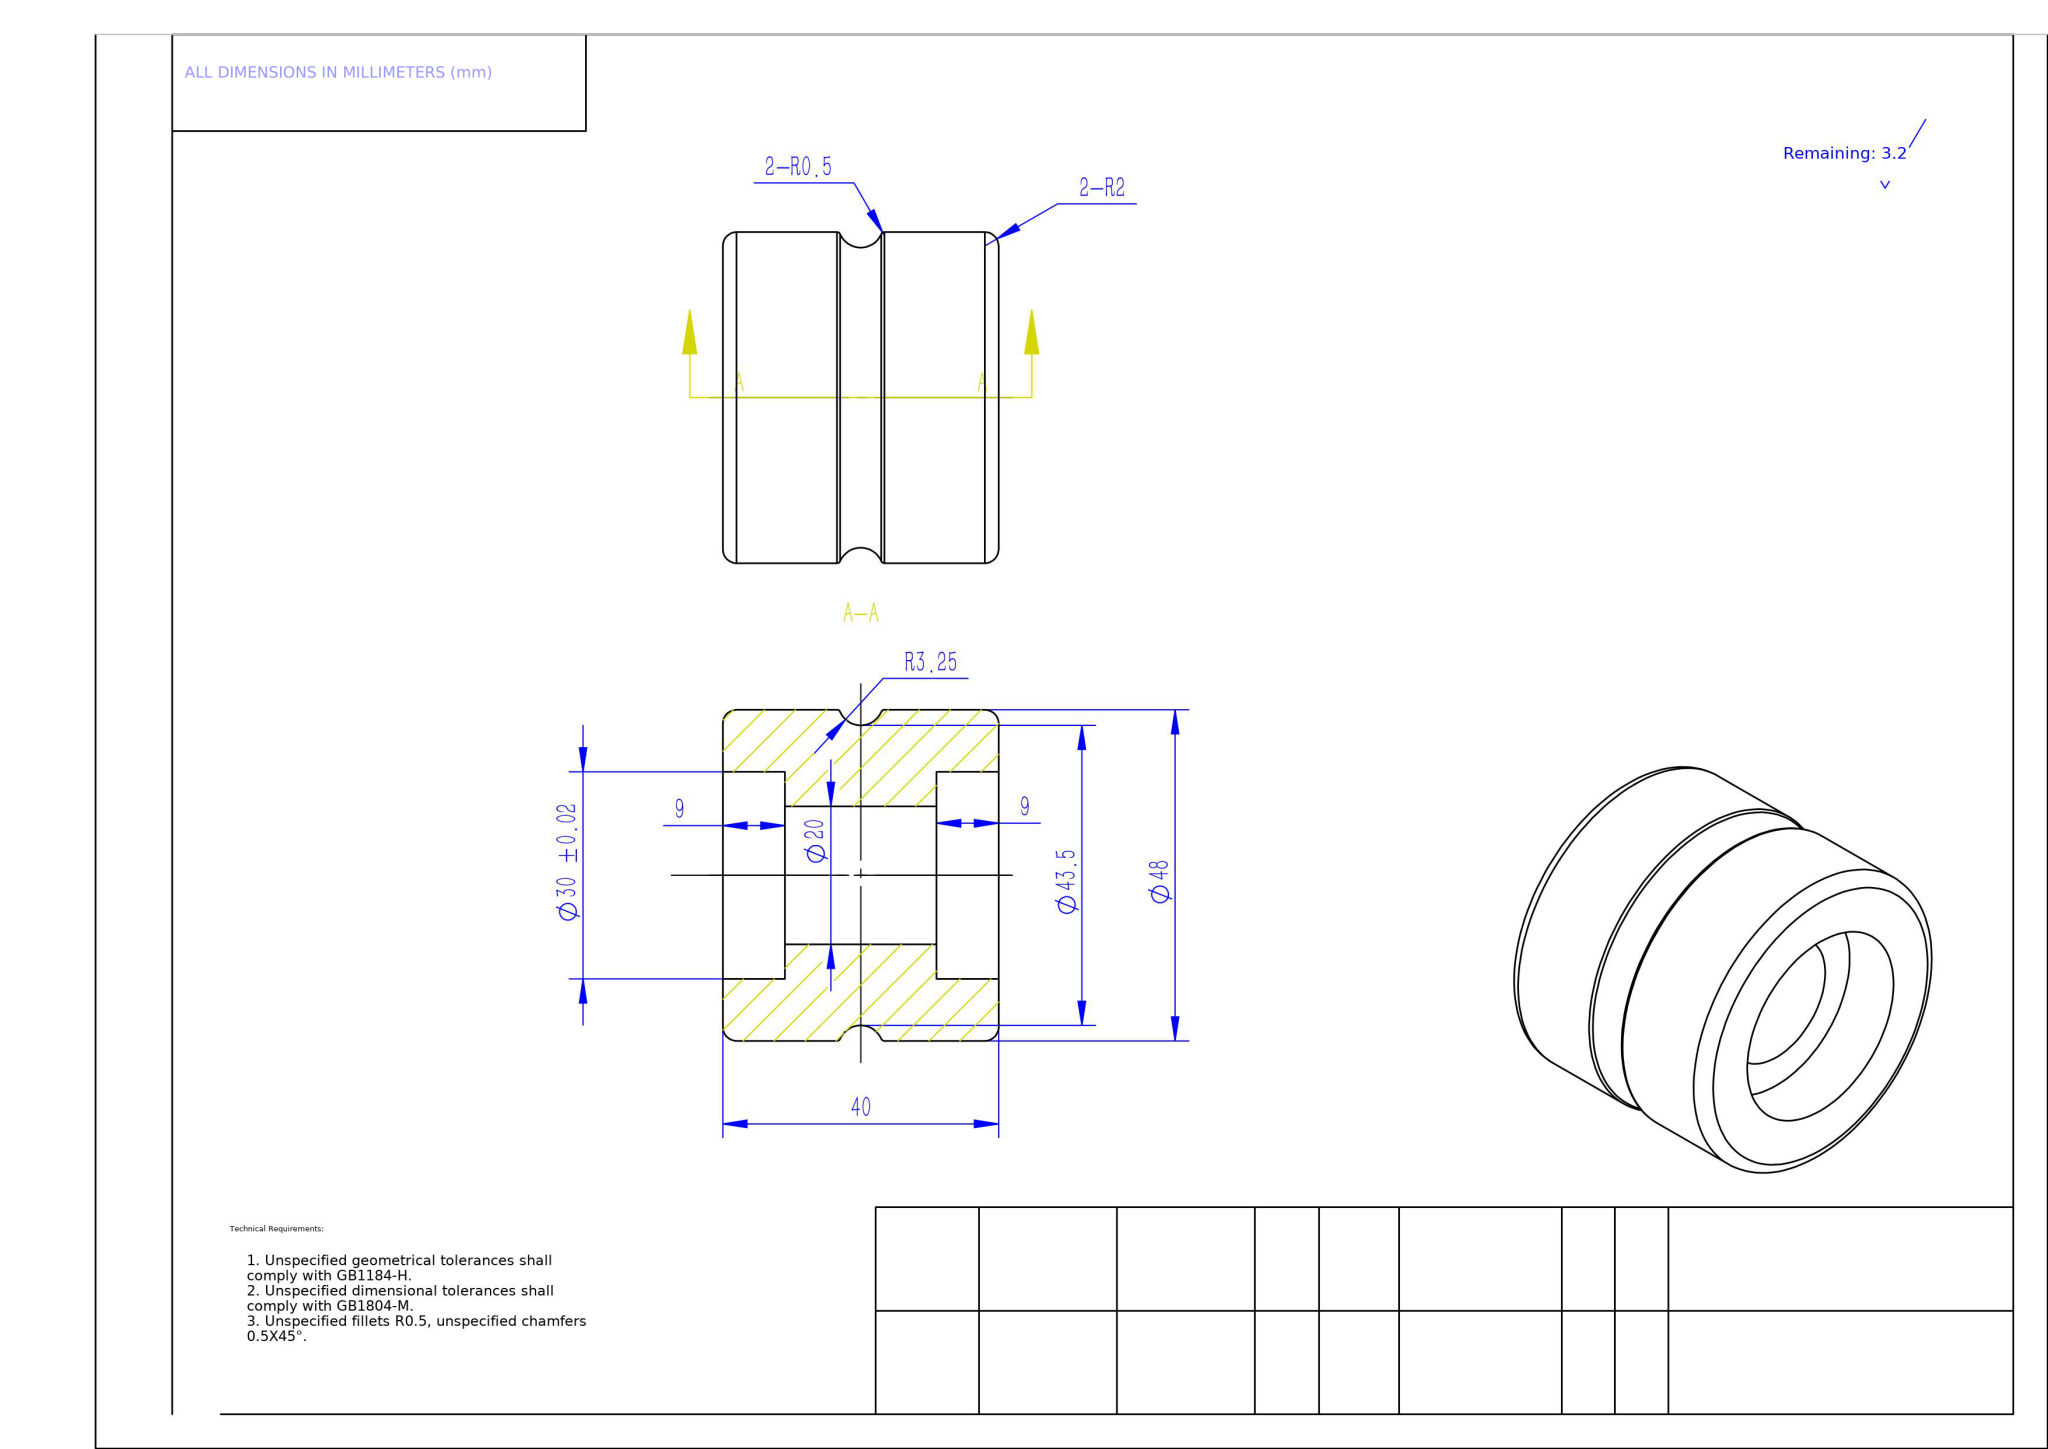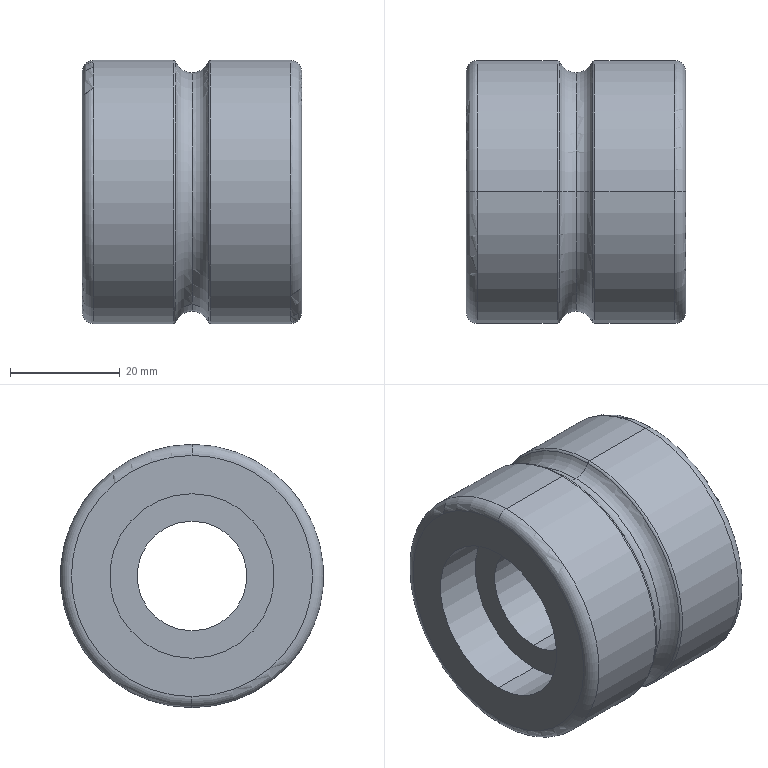Part | NX | mm | 1 solid | 26 faces | box 40 x 48 x 48 mm | volume 51009 mm3 | torus 12 | cylinder 10 | plane 4 | commonest cylinder face diameters 30 x4 48 x4 20 x2
STEP:
#1=COLOUR_RGB('',0.5294,0.549,0.549);
#2=FILL_AREA_STYLE_COLOUR('',#1);
#3=FILL_AREA_STYLE('',(#2));
#4=SURFACE_STYLE_FILL_AREA(#3);
#5=SURFACE_SIDE_STYLE('',(#4));
#6=SURFACE_STYLE_USAGE(.BOTH.,#5);
#7=PRESENTATION_STYLE_ASSIGNMENT((#6));
#8=CARTESIAN_POINT('',(17.021,0.,23.7));
#9=VERTEX_POINT('',#8);
#10=CARTESIAN_POINT('',(20.,0.,21.75));
#11=VERTEX_POINT('',#10);
#12=CARTESIAN_POINT('',(20.,0.,25.));
#13=DIRECTION('',(0.,-1.,0.));
#14=DIRECTION('',(0.,0.,-1.));
#15=AXIS2_PLACEMENT_3D('',#12,#13,#14);
#16=CIRCLE('',#15,3.25);
#17=EDGE_CURVE('',#9,#11,#16,.T.);
#18=ORIENTED_EDGE('',*,*,#17,.T.);
#19=CARTESIAN_POINT('',(20.,0.,-21.75));
#20=VERTEX_POINT('',#19);
#21=CARTESIAN_POINT('',(20.,0.,0.));
#22=DIRECTION('',(-1.,0.,0.));
#23=DIRECTION('',(0.,0.,1.));
#24=AXIS2_PLACEMENT_3D('',#21,#22,#23);
#25=CIRCLE('',#24,21.75);
#26=EDGE_CURVE('',#11,#20,#25,.T.);
#27=ORIENTED_EDGE('',*,*,#26,.T.);
#28=CARTESIAN_POINT('',(17.021,0.,-23.7));
#29=VERTEX_POINT('',#28);
#30=CARTESIAN_POINT('',(20.,0.,-25.));
#31=DIRECTION('',(0.,1.,0.));
#32=DIRECTION('',(0.,-0.,1.));
#33=AXIS2_PLACEMENT_3D('',#30,#31,#32);
#34=CIRCLE('',#33,3.25);
#35=EDGE_CURVE('',#29,#20,#34,.T.);
#36=ORIENTED_EDGE('',*,*,#35,.F.);
#37=CARTESIAN_POINT('',(17.021,0.,0.));
#38=DIRECTION('',(1.,0.,0.));
#39=DIRECTION('',(0.,0.,-1.));
#40=AXIS2_PLACEMENT_3D('',#37,#38,#39);
#41=CIRCLE('',#40,23.7);
#42=EDGE_CURVE('',#29,#9,#41,.T.);
#43=ORIENTED_EDGE('',*,*,#42,.T.);
#44=EDGE_LOOP('',(#18,#27,#36,#43));
#45=FACE_OUTER_BOUND('',#44,.T.);
#46=CARTESIAN_POINT('',(20.,0.,0.));
#47=DIRECTION('',(-1.,0.,0.));
#48=DIRECTION('',(0.,0.,1.));
#49=AXIS2_PLACEMENT_3D('',#46,#47,#48);
#50=TOROIDAL_SURFACE('',#49,25.,3.25);
#51=ADVANCED_FACE('',(#45),#50,.F.);
#52=ORIENTED_EDGE('',*,*,#35,.T.);
#53=CARTESIAN_POINT('',(20.,0.,0.));
#54=DIRECTION('',(-1.,0.,0.));
#55=DIRECTION('',(0.,0.,1.));
#56=AXIS2_PLACEMENT_3D('',#53,#54,#55);
#57=CIRCLE('',#56,21.75);
#58=EDGE_CURVE('',#20,#11,#57,.T.);
#59=ORIENTED_EDGE('',*,*,#58,.T.);
#60=ORIENTED_EDGE('',*,*,#17,.F.);
#61=CARTESIAN_POINT('',(17.021,0.,0.));
#62=DIRECTION('',(1.,0.,0.));
#63=DIRECTION('',(0.,0.,-1.));
#64=AXIS2_PLACEMENT_3D('',#61,#62,#63);
#65=CIRCLE('',#64,23.7);
#66=EDGE_CURVE('',#9,#29,#65,.T.);
#67=ORIENTED_EDGE('',*,*,#66,.T.);
#68=EDGE_LOOP('',(#52,#59,#60,#67));
#69=FACE_OUTER_BOUND('',#68,.T.);
#70=CARTESIAN_POINT('',(20.,0.,0.));
#71=DIRECTION('',(-1.,0.,0.));
#72=DIRECTION('',(0.,0.,1.));
#73=AXIS2_PLACEMENT_3D('',#70,#71,#72);
#74=TOROIDAL_SURFACE('',#73,25.,3.25);
#75=ADVANCED_FACE('',(#69),#74,.F.);
#76=CARTESIAN_POINT('',(16.563,0.,24.));
#77=VERTEX_POINT('',#76);
#78=CARTESIAN_POINT('',(16.563,0.,-24.));
#79=VERTEX_POINT('',#78);
#80=CARTESIAN_POINT('',(16.563,0.,0.));
#81=DIRECTION('',(-1.,0.,0.));
#82=DIRECTION('',(0.,0.,-1.));
#83=AXIS2_PLACEMENT_3D('',#80,#81,#82);
#84=CIRCLE('',#83,24.);
#85=EDGE_CURVE('',#77,#79,#84,.T.);
#86=ORIENTED_EDGE('',*,*,#85,.F.);
#87=CARTESIAN_POINT('',(16.563,0.,23.5));
#88=DIRECTION('',(0.,1.,-0.));
#89=DIRECTION('',(0.,0.,1.));
#90=AXIS2_PLACEMENT_3D('',#87,#88,#89);
#91=CIRCLE('',#90,0.5);
#92=EDGE_CURVE('',#77,#9,#91,.T.);
#93=ORIENTED_EDGE('',*,*,#92,.T.);
#94=ORIENTED_EDGE('',*,*,#42,.F.);
#95=CARTESIAN_POINT('',(16.563,0.,-23.5));
#96=DIRECTION('',(0.,-1.,0.));
#97=DIRECTION('',(0.,0.,-1.));
#98=AXIS2_PLACEMENT_3D('',#95,#96,#97);
#99=CIRCLE('',#98,0.5);
#100=EDGE_CURVE('',#79,#29,#99,.T.);
#101=ORIENTED_EDGE('',*,*,#100,.F.);
#102=EDGE_LOOP('',(#86,#93,#94,#101));
#103=FACE_OUTER_BOUND('',#102,.T.);
#104=CARTESIAN_POINT('',(16.563,0.,0.));
#105=DIRECTION('',(1.,0.,0.));
#106=DIRECTION('',(0.,0.,-1.));
#107=AXIS2_PLACEMENT_3D('',#104,#105,#106);
#108=TOROIDAL_SURFACE('',#107,23.5,0.5);
#109=ADVANCED_FACE('',(#103),#108,.T.);
#110=CARTESIAN_POINT('',(22.979,0.,23.7));
#111=VERTEX_POINT('',#110);
#112=CARTESIAN_POINT('',(22.979,0.,-23.7));
#113=VERTEX_POINT('',#112);
#114=CARTESIAN_POINT('',(22.979,0.,0.));
#115=DIRECTION('',(-1.,0.,0.));
#116=DIRECTION('',(0.,0.,1.));
#117=AXIS2_PLACEMENT_3D('',#114,#115,#116);
#118=CIRCLE('',#117,23.7);
#119=EDGE_CURVE('',#111,#113,#118,.T.);
#120=ORIENTED_EDGE('',*,*,#119,.F.);
#121=CARTESIAN_POINT('',(23.437,0.,24.));
#122=VERTEX_POINT('',#121);
#123=CARTESIAN_POINT('',(23.437,0.,23.5));
#124=DIRECTION('',(0.,1.,-0.));
#125=DIRECTION('',(0.,0.,1.));
#126=AXIS2_PLACEMENT_3D('',#123,#124,#125);
#127=CIRCLE('',#126,0.5);
#128=EDGE_CURVE('',#111,#122,#127,.T.);
#129=ORIENTED_EDGE('',*,*,#128,.T.);
#130=CARTESIAN_POINT('',(23.437,0.,-24.));
#131=VERTEX_POINT('',#130);
#132=CARTESIAN_POINT('',(23.437,0.,0.));
#133=DIRECTION('',(1.,0.,0.));
#134=DIRECTION('',(0.,0.,-1.));
#135=AXIS2_PLACEMENT_3D('',#132,#133,#134);
#136=CIRCLE('',#135,24.);
#137=EDGE_CURVE('',#131,#122,#136,.T.);
#138=ORIENTED_EDGE('',*,*,#137,.F.);
#139=CARTESIAN_POINT('',(23.437,0.,-23.5));
#140=DIRECTION('',(0.,-1.,0.));
#141=DIRECTION('',(0.,0.,-1.));
#142=AXIS2_PLACEMENT_3D('',#139,#140,#141);
#143=CIRCLE('',#142,0.5);
#144=EDGE_CURVE('',#113,#131,#143,.T.);
#145=ORIENTED_EDGE('',*,*,#144,.F.);
#146=EDGE_LOOP('',(#120,#129,#138,#145));
#147=FACE_OUTER_BOUND('',#146,.T.);
#148=CARTESIAN_POINT('',(23.437,0.,0.));
#149=DIRECTION('',(1.,0.,0.));
#150=DIRECTION('',(0.,0.,-1.));
#151=AXIS2_PLACEMENT_3D('',#148,#149,#150);
#152=TOROIDAL_SURFACE('',#151,23.5,0.5);
#153=ADVANCED_FACE('',(#147),#152,.T.);
#154=CARTESIAN_POINT('',(2.,0.,-24.));
#155=VERTEX_POINT('',#154);
#156=CARTESIAN_POINT('',(2.,0.,24.));
#157=VERTEX_POINT('',#156);
#158=CARTESIAN_POINT('',(2.,0.,0.));
#159=DIRECTION('',(1.,0.,0.));
#160=DIRECTION('',(0.,0.,1.));
#161=AXIS2_PLACEMENT_3D('',#158,#159,#160);
#162=CIRCLE('',#161,24.);
#163=EDGE_CURVE('',#155,#157,#162,.T.);
#164=ORIENTED_EDGE('',*,*,#163,.F.);
#165=CARTESIAN_POINT('',(-0.,0.,-22.));
#166=VERTEX_POINT('',#165);
#167=CARTESIAN_POINT('',(2.,0.,-22.));
#168=DIRECTION('',(0.,1.,0.));
#169=DIRECTION('',(0.,-0.,1.));
#170=AXIS2_PLACEMENT_3D('',#167,#168,#169);
#171=CIRCLE('',#170,2.);
#172=EDGE_CURVE('',#155,#166,#171,.T.);
#173=ORIENTED_EDGE('',*,*,#172,.T.);
#174=CARTESIAN_POINT('',(-0.,0.,22.));
#175=VERTEX_POINT('',#174);
#176=CARTESIAN_POINT('',(-0.,0.,0.));
#177=DIRECTION('',(-1.,0.,0.));
#178=DIRECTION('',(0.,0.,1.));
#179=AXIS2_PLACEMENT_3D('',#176,#177,#178);
#180=CIRCLE('',#179,22.);
#181=EDGE_CURVE('',#175,#166,#180,.T.);
#182=ORIENTED_EDGE('',*,*,#181,.F.);
#183=CARTESIAN_POINT('',(2.,0.,22.));
#184=DIRECTION('',(0.,-1.,0.));
#185=DIRECTION('',(0.,0.,-1.));
#186=AXIS2_PLACEMENT_3D('',#183,#184,#185);
#187=CIRCLE('',#186,2.);
#188=EDGE_CURVE('',#157,#175,#187,.T.);
#189=ORIENTED_EDGE('',*,*,#188,.F.);
#190=EDGE_LOOP('',(#164,#173,#182,#189));
#191=FACE_OUTER_BOUND('',#190,.T.);
#192=CARTESIAN_POINT('',(2.,0.,0.));
#193=DIRECTION('',(-1.,0.,0.));
#194=DIRECTION('',(0.,0.,1.));
#195=AXIS2_PLACEMENT_3D('',#192,#193,#194);
#196=TOROIDAL_SURFACE('',#195,22.,2.);
#197=ADVANCED_FACE('',(#191),#196,.T.);
#198=CARTESIAN_POINT('',(38.,0.,24.));
#199=VERTEX_POINT('',#198);
#200=CARTESIAN_POINT('',(38.,0.,-24.));
#201=VERTEX_POINT('',#200);
#202=CARTESIAN_POINT('',(38.,0.,0.));
#203=DIRECTION('',(-1.,0.,0.));
#204=DIRECTION('',(0.,0.,-1.));
#205=AXIS2_PLACEMENT_3D('',#202,#203,#204);
#206=CIRCLE('',#205,24.);
#207=EDGE_CURVE('',#199,#201,#206,.T.);
#208=ORIENTED_EDGE('',*,*,#207,.F.);
#209=CARTESIAN_POINT('',(40.,0.,22.));
#210=VERTEX_POINT('',#209);
#211=CARTESIAN_POINT('',(38.,0.,22.));
#212=DIRECTION('',(0.,1.,-0.));
#213=DIRECTION('',(0.,0.,1.));
#214=AXIS2_PLACEMENT_3D('',#211,#212,#213);
#215=CIRCLE('',#214,2.);
#216=EDGE_CURVE('',#199,#210,#215,.T.);
#217=ORIENTED_EDGE('',*,*,#216,.T.);
#218=CARTESIAN_POINT('',(40.,0.,-22.));
#219=VERTEX_POINT('',#218);
#220=CARTESIAN_POINT('',(40.,0.,0.));
#221=DIRECTION('',(1.,0.,0.));
#222=DIRECTION('',(0.,0.,-1.));
#223=AXIS2_PLACEMENT_3D('',#220,#221,#222);
#224=CIRCLE('',#223,22.);
#225=EDGE_CURVE('',#219,#210,#224,.T.);
#226=ORIENTED_EDGE('',*,*,#225,.F.);
#227=CARTESIAN_POINT('',(38.,0.,-22.));
#228=DIRECTION('',(0.,-1.,0.));
#229=DIRECTION('',(0.,0.,-1.));
#230=AXIS2_PLACEMENT_3D('',#227,#228,#229);
#231=CIRCLE('',#230,2.);
#232=EDGE_CURVE('',#201,#219,#231,.T.);
#233=ORIENTED_EDGE('',*,*,#232,.F.);
#234=EDGE_LOOP('',(#208,#217,#226,#233));
#235=FACE_OUTER_BOUND('',#234,.T.);
#236=CARTESIAN_POINT('',(38.,0.,0.));
#237=DIRECTION('',(1.,0.,0.));
#238=DIRECTION('',(0.,0.,-1.));
#239=AXIS2_PLACEMENT_3D('',#236,#237,#238);
#240=TOROIDAL_SURFACE('',#239,22.,2.);
#241=ADVANCED_FACE('',(#235),#240,.T.);
#242=CARTESIAN_POINT('',(40.,0.,-15.));
#243=VERTEX_POINT('',#242);
#244=CARTESIAN_POINT('',(40.,0.,15.));
#245=VERTEX_POINT('',#244);
#246=CARTESIAN_POINT('',(40.,0.,0.));
#247=DIRECTION('',(-1.,0.,0.));
#248=DIRECTION('',(0.,0.,1.));
#249=AXIS2_PLACEMENT_3D('',#246,#247,#248);
#250=CIRCLE('',#249,15.);
#251=EDGE_CURVE('',#243,#245,#250,.T.);
#252=ORIENTED_EDGE('',*,*,#251,.F.);
#253=CARTESIAN_POINT('',(31.,0.,-15.));
#254=VERTEX_POINT('',#253);
#255=CARTESIAN_POINT('',(0.,0.,-15.));
#256=DIRECTION('',(-1.,0.,0.));
#257=VECTOR('',#256,1000.);
#258=LINE('',#255,#257);
#259=EDGE_CURVE('',#243,#254,#258,.T.);
#260=ORIENTED_EDGE('',*,*,#259,.T.);
#261=CARTESIAN_POINT('',(31.,0.,15.));
#262=VERTEX_POINT('',#261);
#263=CARTESIAN_POINT('',(31.,0.,0.));
#264=DIRECTION('',(-1.,0.,0.));
#265=DIRECTION('',(0.,0.,1.));
#266=AXIS2_PLACEMENT_3D('',#263,#264,#265);
#267=CIRCLE('',#266,15.);
#268=EDGE_CURVE('',#254,#262,#267,.T.);
#269=ORIENTED_EDGE('',*,*,#268,.T.);
#270=CARTESIAN_POINT('',(0.,0.,15.));
#271=DIRECTION('',(-1.,0.,0.));
#272=VECTOR('',#271,1000.);
#273=LINE('',#270,#272);
#274=EDGE_CURVE('',#245,#262,#273,.T.);
#275=ORIENTED_EDGE('',*,*,#274,.F.);
#276=EDGE_LOOP('',(#252,#260,#269,#275));
#277=FACE_OUTER_BOUND('',#276,.T.);
#278=CARTESIAN_POINT('',(0.,0.,0.));
#279=DIRECTION('',(-1.,0.,0.));
#280=DIRECTION('',(0.,0.,1.));
#281=AXIS2_PLACEMENT_3D('',#278,#279,#280);
#282=CYLINDRICAL_SURFACE('',#281,15.);
#283=ADVANCED_FACE('',(#277),#282,.F.);
#284=CARTESIAN_POINT('',(31.,0.,-10.));
#285=VERTEX_POINT('',#284);
#286=CARTESIAN_POINT('',(31.,0.,10.));
#287=VERTEX_POINT('',#286);
#288=CARTESIAN_POINT('',(31.,0.,0.));
#289=DIRECTION('',(-1.,0.,0.));
#290=DIRECTION('',(0.,0.,1.));
#291=AXIS2_PLACEMENT_3D('',#288,#289,#290);
#292=CIRCLE('',#291,10.);
#293=EDGE_CURVE('',#285,#287,#292,.T.);
#294=ORIENTED_EDGE('',*,*,#293,.F.);
#295=CARTESIAN_POINT('',(9.,0.,-10.));
#296=VERTEX_POINT('',#295);
#297=CARTESIAN_POINT('',(0.,0.,-10.));
#298=DIRECTION('',(-1.,0.,0.));
#299=VECTOR('',#298,1000.);
#300=LINE('',#297,#299);
#301=EDGE_CURVE('',#285,#296,#300,.T.);
#302=ORIENTED_EDGE('',*,*,#301,.T.);
#303=CARTESIAN_POINT('',(9.,0.,10.));
#304=VERTEX_POINT('',#303);
#305=CARTESIAN_POINT('',(9.,0.,0.));
#306=DIRECTION('',(-1.,0.,0.));
#307=DIRECTION('',(0.,0.,1.));
#308=AXIS2_PLACEMENT_3D('',#305,#306,#307);
#309=CIRCLE('',#308,10.);
#310=EDGE_CURVE('',#296,#304,#309,.T.);
#311=ORIENTED_EDGE('',*,*,#310,.T.);
#312=CARTESIAN_POINT('',(0.,0.,10.));
#313=DIRECTION('',(-1.,0.,0.));
#314=VECTOR('',#313,1000.);
#315=LINE('',#312,#314);
#316=EDGE_CURVE('',#287,#304,#315,.T.);
#317=ORIENTED_EDGE('',*,*,#316,.F.);
#318=EDGE_LOOP('',(#294,#302,#311,#317));
#319=FACE_OUTER_BOUND('',#318,.T.);
#320=CARTESIAN_POINT('',(0.,0.,0.));
#321=DIRECTION('',(-1.,0.,0.));
#322=DIRECTION('',(0.,0.,1.));
#323=AXIS2_PLACEMENT_3D('',#320,#321,#322);
#324=CYLINDRICAL_SURFACE('',#323,10.);
#325=ADVANCED_FACE('',(#319),#324,.F.);
#326=CARTESIAN_POINT('',(9.,0.,-15.));
#327=VERTEX_POINT('',#326);
#328=CARTESIAN_POINT('',(9.,0.,15.));
#329=VERTEX_POINT('',#328);
#330=CARTESIAN_POINT('',(9.,0.,0.));
#331=DIRECTION('',(-1.,0.,0.));
#332=DIRECTION('',(0.,0.,1.));
#333=AXIS2_PLACEMENT_3D('',#330,#331,#332);
#334=CIRCLE('',#333,15.);
#335=EDGE_CURVE('',#327,#329,#334,.T.);
#336=ORIENTED_EDGE('',*,*,#335,.F.);
#337=CARTESIAN_POINT('',(0.,0.,-15.));
#338=VERTEX_POINT('',#337);
#339=CARTESIAN_POINT('',(0.,0.,-15.));
#340=DIRECTION('',(-1.,0.,0.));
#341=VECTOR('',#340,1000.);
#342=LINE('',#339,#341);
#343=EDGE_CURVE('',#327,#338,#342,.T.);
#344=ORIENTED_EDGE('',*,*,#343,.T.);
#345=CARTESIAN_POINT('',(0.,0.,15.));
#346=VERTEX_POINT('',#345);
#347=CARTESIAN_POINT('',(0.,0.,0.));
#348=DIRECTION('',(-1.,0.,0.));
#349=DIRECTION('',(0.,0.,1.));
#350=AXIS2_PLACEMENT_3D('',#347,#348,#349);
#351=CIRCLE('',#350,15.);
#352=EDGE_CURVE('',#338,#346,#351,.T.);
#353=ORIENTED_EDGE('',*,*,#352,.T.);
#354=CARTESIAN_POINT('',(0.,0.,15.));
#355=DIRECTION('',(-1.,0.,0.));
#356=VECTOR('',#355,1000.);
#357=LINE('',#354,#356);
#358=EDGE_CURVE('',#329,#346,#357,.T.);
#359=ORIENTED_EDGE('',*,*,#358,.F.);
#360=EDGE_LOOP('',(#336,#344,#353,#359));
#361=FACE_OUTER_BOUND('',#360,.T.);
#362=CARTESIAN_POINT('',(0.,0.,0.));
#363=DIRECTION('',(-1.,0.,0.));
#364=DIRECTION('',(0.,0.,1.));
#365=AXIS2_PLACEMENT_3D('',#362,#363,#364);
#366=CYLINDRICAL_SURFACE('',#365,15.);
#367=ADVANCED_FACE('',(#361),#366,.F.);
#368=ORIENTED_EDGE('',*,*,#85,.T.);
#369=CARTESIAN_POINT('',(0.,0.,-24.));
#370=DIRECTION('',(-1.,0.,0.));
#371=VECTOR('',#370,1000.);
#372=LINE('',#369,#371);
#373=EDGE_CURVE('',#79,#155,#372,.T.);
#374=ORIENTED_EDGE('',*,*,#373,.T.);
#375=ORIENTED_EDGE('',*,*,#163,.T.);
#376=CARTESIAN_POINT('',(0.,0.,24.));
#377=DIRECTION('',(-1.,0.,0.));
#378=VECTOR('',#377,1000.);
#379=LINE('',#376,#378);
#380=EDGE_CURVE('',#77,#157,#379,.T.);
#381=ORIENTED_EDGE('',*,*,#380,.F.);
#382=EDGE_LOOP('',(#368,#374,#375,#381));
#383=FACE_OUTER_BOUND('',#382,.T.);
#384=CARTESIAN_POINT('',(0.,0.,0.));
#385=DIRECTION('',(-1.,0.,0.));
#386=DIRECTION('',(0.,0.,1.));
#387=AXIS2_PLACEMENT_3D('',#384,#385,#386);
#388=CYLINDRICAL_SURFACE('',#387,24.);
#389=ADVANCED_FACE('',(#383),#388,.T.);
#390=ORIENTED_EDGE('',*,*,#58,.F.);
#391=CARTESIAN_POINT('',(20.,0.,-25.));
#392=DIRECTION('',(0.,1.,0.));
#393=DIRECTION('',(0.,-0.,1.));
#394=AXIS2_PLACEMENT_3D('',#391,#392,#393);
#395=CIRCLE('',#394,3.25);
#396=EDGE_CURVE('',#20,#113,#395,.T.);
#397=ORIENTED_EDGE('',*,*,#396,.T.);
#398=CARTESIAN_POINT('',(22.979,0.,0.));
#399=DIRECTION('',(-1.,0.,0.));
#400=DIRECTION('',(0.,0.,1.));
#401=AXIS2_PLACEMENT_3D('',#398,#399,#400);
#402=CIRCLE('',#401,23.7);
#403=EDGE_CURVE('',#113,#111,#402,.T.);
#404=ORIENTED_EDGE('',*,*,#403,.T.);
#405=CARTESIAN_POINT('',(20.,0.,25.));
#406=DIRECTION('',(0.,-1.,0.));
#407=DIRECTION('',(0.,0.,-1.));
#408=AXIS2_PLACEMENT_3D('',#405,#406,#407);
#409=CIRCLE('',#408,3.25);
#410=EDGE_CURVE('',#11,#111,#409,.T.);
#411=ORIENTED_EDGE('',*,*,#410,.F.);
#412=EDGE_LOOP('',(#390,#397,#404,#411));
#413=FACE_OUTER_BOUND('',#412,.T.);
#414=CARTESIAN_POINT('',(20.,0.,0.));
#415=DIRECTION('',(-1.,0.,0.));
#416=DIRECTION('',(0.,0.,1.));
#417=AXIS2_PLACEMENT_3D('',#414,#415,#416);
#418=TOROIDAL_SURFACE('',#417,25.,3.25);
#419=ADVANCED_FACE('',(#413),#418,.F.);
#420=ORIENTED_EDGE('',*,*,#207,.T.);
#421=CARTESIAN_POINT('',(0.,0.,-24.));
#422=DIRECTION('',(-1.,0.,0.));
#423=VECTOR('',#422,1000.);
#424=LINE('',#421,#423);
#425=EDGE_CURVE('',#201,#131,#424,.T.);
#426=ORIENTED_EDGE('',*,*,#425,.T.);
#427=ORIENTED_EDGE('',*,*,#137,.T.);
#428=CARTESIAN_POINT('',(0.,0.,24.));
#429=DIRECTION('',(-1.,0.,0.));
#430=VECTOR('',#429,1000.);
#431=LINE('',#428,#430);
#432=EDGE_CURVE('',#199,#122,#431,.T.);
#433=ORIENTED_EDGE('',*,*,#432,.F.);
#434=EDGE_LOOP('',(#420,#426,#427,#433));
#435=FACE_OUTER_BOUND('',#434,.T.);
#436=CARTESIAN_POINT('',(0.,0.,0.));
#437=DIRECTION('',(-1.,0.,0.));
#438=DIRECTION('',(0.,0.,1.));
#439=AXIS2_PLACEMENT_3D('',#436,#437,#438);
#440=CYLINDRICAL_SURFACE('',#439,24.);
#441=ADVANCED_FACE('',(#435),#440,.T.);
#442=ORIENTED_EDGE('',*,*,#425,.F.);
#443=CARTESIAN_POINT('',(38.,0.,0.));
#444=DIRECTION('',(-1.,0.,0.));
#445=DIRECTION('',(0.,0.,-1.));
#446=AXIS2_PLACEMENT_3D('',#443,#444,#445);
#447=CIRCLE('',#446,24.);
#448=EDGE_CURVE('',#201,#199,#447,.T.);
#449=ORIENTED_EDGE('',*,*,#448,.T.);
#450=ORIENTED_EDGE('',*,*,#432,.T.);
#451=CARTESIAN_POINT('',(23.437,0.,0.));
#452=DIRECTION('',(1.,0.,0.));
#453=DIRECTION('',(0.,0.,-1.));
#454=AXIS2_PLACEMENT_3D('',#451,#452,#453);
#455=CIRCLE('',#454,24.);
#456=EDGE_CURVE('',#122,#131,#455,.T.);
#457=ORIENTED_EDGE('',*,*,#456,.T.);
#458=EDGE_LOOP('',(#442,#449,#450,#457));
#459=FACE_OUTER_BOUND('',#458,.T.);
#460=CARTESIAN_POINT('',(0.,0.,0.));
#461=DIRECTION('',(-1.,0.,0.));
#462=DIRECTION('',(0.,0.,1.));
#463=AXIS2_PLACEMENT_3D('',#460,#461,#462);
#464=CYLINDRICAL_SURFACE('',#463,24.);
#465=ADVANCED_FACE('',(#459),#464,.T.);
#466=ORIENTED_EDGE('',*,*,#26,.F.);
#467=ORIENTED_EDGE('',*,*,#410,.T.);
#468=ORIENTED_EDGE('',*,*,#119,.T.);
#469=ORIENTED_EDGE('',*,*,#396,.F.);
#470=EDGE_LOOP('',(#466,#467,#468,#469));
#471=FACE_OUTER_BOUND('',#470,.T.);
#472=CARTESIAN_POINT('',(20.,0.,0.));
#473=DIRECTION('',(-1.,0.,0.));
#474=DIRECTION('',(0.,0.,1.));
#475=AXIS2_PLACEMENT_3D('',#472,#473,#474);
#476=TOROIDAL_SURFACE('',#475,25.,3.25);
#477=ADVANCED_FACE('',(#471),#476,.F.);
#478=ORIENTED_EDGE('',*,*,#373,.F.);
#479=CARTESIAN_POINT('',(16.563,0.,0.));
#480=DIRECTION('',(-1.,0.,0.));
#481=DIRECTION('',(0.,0.,-1.));
#482=AXIS2_PLACEMENT_3D('',#479,#480,#481);
#483=CIRCLE('',#482,24.);
#484=EDGE_CURVE('',#79,#77,#483,.T.);
#485=ORIENTED_EDGE('',*,*,#484,.T.);
#486=ORIENTED_EDGE('',*,*,#380,.T.);
#487=CARTESIAN_POINT('',(2.,0.,0.));
#488=DIRECTION('',(1.,0.,0.));
#489=DIRECTION('',(0.,0.,1.));
#490=AXIS2_PLACEMENT_3D('',#487,#488,#489);
#491=CIRCLE('',#490,24.);
#492=EDGE_CURVE('',#157,#155,#491,.T.);
#493=ORIENTED_EDGE('',*,*,#492,.T.);
#494=EDGE_LOOP('',(#478,#485,#486,#493));
#495=FACE_OUTER_BOUND('',#494,.T.);
#496=CARTESIAN_POINT('',(0.,0.,0.));
#497=DIRECTION('',(-1.,0.,0.));
#498=DIRECTION('',(0.,0.,1.));
#499=AXIS2_PLACEMENT_3D('',#496,#497,#498);
#500=CYLINDRICAL_SURFACE('',#499,24.);
#501=ADVANCED_FACE('',(#495),#500,.T.);
#502=ORIENTED_EDGE('',*,*,#181,.T.);
#503=CARTESIAN_POINT('',(-0.,0.,0.));
#504=DIRECTION('',(-1.,0.,0.));
#505=DIRECTION('',(0.,0.,1.));
#506=AXIS2_PLACEMENT_3D('',#503,#504,#505);
#507=CIRCLE('',#506,22.);
#508=EDGE_CURVE('',#166,#175,#507,.T.);
#509=ORIENTED_EDGE('',*,*,#508,.T.);
#510=EDGE_LOOP('',(#502,#509));
#511=FACE_OUTER_BOUND('',#510,.T.);
#512=CARTESIAN_POINT('',(0.,0.,0.));
#513=DIRECTION('',(-1.,0.,0.));
#514=DIRECTION('',(0.,0.,1.));
#515=AXIS2_PLACEMENT_3D('',#512,#513,#514);
#516=CIRCLE('',#515,15.);
#517=EDGE_CURVE('',#346,#338,#516,.T.);
#518=ORIENTED_EDGE('',*,*,#517,.F.);
#519=ORIENTED_EDGE('',*,*,#352,.F.);
#520=EDGE_LOOP('',(#518,#519));
#521=FACE_BOUND('',#520,.T.);
#522=CARTESIAN_POINT('',(-0.,-15.,0.));
#523=DIRECTION('',(-1.,0.,0.));
#524=DIRECTION('',(0.,0.,1.));
#525=AXIS2_PLACEMENT_3D('',#522,#523,#524);
#526=PLANE('',#525);
#527=ADVANCED_FACE('',(#511,#521),#526,.T.);
#528=ORIENTED_EDGE('',*,*,#343,.F.);
#529=CARTESIAN_POINT('',(9.,0.,0.));
#530=DIRECTION('',(-1.,0.,0.));
#531=DIRECTION('',(0.,0.,1.));
#532=AXIS2_PLACEMENT_3D('',#529,#530,#531);
#533=CIRCLE('',#532,15.);
#534=EDGE_CURVE('',#329,#327,#533,.T.);
#535=ORIENTED_EDGE('',*,*,#534,.F.);
#536=ORIENTED_EDGE('',*,*,#358,.T.);
#537=ORIENTED_EDGE('',*,*,#517,.T.);
#538=EDGE_LOOP('',(#528,#535,#536,#537));
#539=FACE_OUTER_BOUND('',#538,.T.);
#540=CARTESIAN_POINT('',(0.,0.,0.));
#541=DIRECTION('',(-1.,0.,0.));
#542=DIRECTION('',(0.,0.,1.));
#543=AXIS2_PLACEMENT_3D('',#540,#541,#542);
#544=CYLINDRICAL_SURFACE('',#543,15.);
#545=ADVANCED_FACE('',(#539),#544,.F.);
#546=ORIENTED_EDGE('',*,*,#534,.T.);
#547=ORIENTED_EDGE('',*,*,#335,.T.);
#548=EDGE_LOOP('',(#546,#547));
#549=FACE_OUTER_BOUND('',#548,.T.);
#550=CARTESIAN_POINT('',(9.,0.,0.));
#551=DIRECTION('',(-1.,0.,0.));
#552=DIRECTION('',(0.,0.,1.));
#553=AXIS2_PLACEMENT_3D('',#550,#551,#552);
#554=CIRCLE('',#553,10.);
#555=EDGE_CURVE('',#304,#296,#554,.T.);
#556=ORIENTED_EDGE('',*,*,#555,.F.);
#557=ORIENTED_EDGE('',*,*,#310,.F.);
#558=EDGE_LOOP('',(#556,#557));
#559=FACE_BOUND('',#558,.T.);
#560=CARTESIAN_POINT('',(9.,-10.,0.));
#561=DIRECTION('',(-1.,0.,0.));
#562=DIRECTION('',(0.,0.,1.));
#563=AXIS2_PLACEMENT_3D('',#560,#561,#562);
#564=PLANE('',#563);
#565=ADVANCED_FACE('',(#549,#559),#564,.T.);
#566=ORIENTED_EDGE('',*,*,#301,.F.);
#567=CARTESIAN_POINT('',(31.,0.,0.));
#568=DIRECTION('',(-1.,0.,0.));
#569=DIRECTION('',(0.,0.,1.));
#570=AXIS2_PLACEMENT_3D('',#567,#568,#569);
#571=CIRCLE('',#570,10.);
#572=EDGE_CURVE('',#287,#285,#571,.T.);
#573=ORIENTED_EDGE('',*,*,#572,.F.);
#574=ORIENTED_EDGE('',*,*,#316,.T.);
#575=ORIENTED_EDGE('',*,*,#555,.T.);
#576=EDGE_LOOP('',(#566,#573,#574,#575));
#577=FACE_OUTER_BOUND('',#576,.T.);
#578=CARTESIAN_POINT('',(0.,0.,0.));
#579=DIRECTION('',(-1.,0.,0.));
#580=DIRECTION('',(0.,0.,1.));
#581=AXIS2_PLACEMENT_3D('',#578,#579,#580);
#582=CYLINDRICAL_SURFACE('',#581,10.);
#583=ADVANCED_FACE('',(#577),#582,.F.);
#584=ORIENTED_EDGE('',*,*,#572,.T.);
#585=ORIENTED_EDGE('',*,*,#293,.T.);
#586=EDGE_LOOP('',(#584,#585));
#587=FACE_BOUND('',#586,.T.);
#588=CARTESIAN_POINT('',(31.,0.,0.));
#589=DIRECTION('',(-1.,0.,0.));
#590=DIRECTION('',(0.,0.,1.));
#591=AXIS2_PLACEMENT_3D('',#588,#589,#590);
#592=CIRCLE('',#591,15.);
#593=EDGE_CURVE('',#262,#254,#592,.T.);
#594=ORIENTED_EDGE('',*,*,#593,.F.);
#595=ORIENTED_EDGE('',*,*,#268,.F.);
#596=EDGE_LOOP('',(#594,#595));
#597=FACE_OUTER_BOUND('',#596,.T.);
#598=CARTESIAN_POINT('',(31.,-15.,0.));
#599=DIRECTION('',(1.,0.,0.));
#600=DIRECTION('',(0.,0.,-1.));
#601=AXIS2_PLACEMENT_3D('',#598,#599,#600);
#602=PLANE('',#601);
#603=ADVANCED_FACE('',(#587,#597),#602,.T.);
#604=ORIENTED_EDGE('',*,*,#259,.F.);
#605=CARTESIAN_POINT('',(40.,0.,0.));
#606=DIRECTION('',(-1.,0.,0.));
#607=DIRECTION('',(0.,0.,1.));
#608=AXIS2_PLACEMENT_3D('',#605,#606,#607);
#609=CIRCLE('',#608,15.);
#610=EDGE_CURVE('',#245,#243,#609,.T.);
#611=ORIENTED_EDGE('',*,*,#610,.F.);
#612=ORIENTED_EDGE('',*,*,#274,.T.);
#613=ORIENTED_EDGE('',*,*,#593,.T.);
#614=EDGE_LOOP('',(#604,#611,#612,#613));
#615=FACE_OUTER_BOUND('',#614,.T.);
#616=CARTESIAN_POINT('',(0.,0.,0.));
#617=DIRECTION('',(-1.,0.,0.));
#618=DIRECTION('',(0.,0.,1.));
#619=AXIS2_PLACEMENT_3D('',#616,#617,#618);
#620=CYLINDRICAL_SURFACE('',#619,15.);
#621=ADVANCED_FACE('',(#615),#620,.F.);
#622=ORIENTED_EDGE('',*,*,#225,.T.);
#623=CARTESIAN_POINT('',(40.,0.,0.));
#624=DIRECTION('',(1.,0.,0.));
#625=DIRECTION('',(0.,0.,-1.));
#626=AXIS2_PLACEMENT_3D('',#623,#624,#625);
#627=CIRCLE('',#626,22.);
#628=EDGE_CURVE('',#210,#219,#627,.T.);
#629=ORIENTED_EDGE('',*,*,#628,.T.);
#630=EDGE_LOOP('',(#622,#629));
#631=FACE_OUTER_BOUND('',#630,.T.);
#632=ORIENTED_EDGE('',*,*,#610,.T.);
#633=ORIENTED_EDGE('',*,*,#251,.T.);
#634=EDGE_LOOP('',(#632,#633));
#635=FACE_BOUND('',#634,.T.);
#636=CARTESIAN_POINT('',(40.,-24.,0.));
#637=DIRECTION('',(1.,0.,0.));
#638=DIRECTION('',(0.,0.,-1.));
#639=AXIS2_PLACEMENT_3D('',#636,#637,#638);
#640=PLANE('',#639);
#641=ADVANCED_FACE('',(#631,#635),#640,.T.);
#642=ORIENTED_EDGE('',*,*,#216,.F.);
#643=ORIENTED_EDGE('',*,*,#448,.F.);
#644=ORIENTED_EDGE('',*,*,#232,.T.);
#645=ORIENTED_EDGE('',*,*,#628,.F.);
#646=EDGE_LOOP('',(#642,#643,#644,#645));
#647=FACE_OUTER_BOUND('',#646,.T.);
#648=CARTESIAN_POINT('',(38.,0.,0.));
#649=DIRECTION('',(1.,0.,0.));
#650=DIRECTION('',(0.,0.,-1.));
#651=AXIS2_PLACEMENT_3D('',#648,#649,#650);
#652=TOROIDAL_SURFACE('',#651,22.,2.);
#653=ADVANCED_FACE('',(#647),#652,.T.);
#654=ORIENTED_EDGE('',*,*,#172,.F.);
#655=ORIENTED_EDGE('',*,*,#492,.F.);
#656=ORIENTED_EDGE('',*,*,#188,.T.);
#657=ORIENTED_EDGE('',*,*,#508,.F.);
#658=EDGE_LOOP('',(#654,#655,#656,#657));
#659=FACE_OUTER_BOUND('',#658,.T.);
#660=CARTESIAN_POINT('',(2.,0.,0.));
#661=DIRECTION('',(-1.,0.,0.));
#662=DIRECTION('',(0.,0.,1.));
#663=AXIS2_PLACEMENT_3D('',#660,#661,#662);
#664=TOROIDAL_SURFACE('',#663,22.,2.);
#665=ADVANCED_FACE('',(#659),#664,.T.);
#666=ORIENTED_EDGE('',*,*,#128,.F.);
#667=ORIENTED_EDGE('',*,*,#403,.F.);
#668=ORIENTED_EDGE('',*,*,#144,.T.);
#669=ORIENTED_EDGE('',*,*,#456,.F.);
#670=EDGE_LOOP('',(#666,#667,#668,#669));
#671=FACE_OUTER_BOUND('',#670,.T.);
#672=CARTESIAN_POINT('',(23.437,0.,0.));
#673=DIRECTION('',(1.,0.,0.));
#674=DIRECTION('',(0.,0.,-1.));
#675=AXIS2_PLACEMENT_3D('',#672,#673,#674);
#676=TOROIDAL_SURFACE('',#675,23.5,0.5);
#677=ADVANCED_FACE('',(#671),#676,.T.);
#678=ORIENTED_EDGE('',*,*,#92,.F.);
#679=ORIENTED_EDGE('',*,*,#484,.F.);
#680=ORIENTED_EDGE('',*,*,#100,.T.);
#681=ORIENTED_EDGE('',*,*,#66,.F.);
#682=EDGE_LOOP('',(#678,#679,#680,#681));
#683=FACE_OUTER_BOUND('',#682,.T.);
#684=CARTESIAN_POINT('',(16.563,0.,0.));
#685=DIRECTION('',(1.,0.,0.));
#686=DIRECTION('',(0.,0.,-1.));
#687=AXIS2_PLACEMENT_3D('',#684,#685,#686);
#688=TOROIDAL_SURFACE('',#687,23.5,0.5);
#689=ADVANCED_FACE('',(#683),#688,.T.);
#690=CLOSED_SHELL('',(#51,#75,#109,#153,#197,#241,#283,#325,#367,#389,#419,#441,#465,#477,#501,#527,#545,#565,#583,#603,#621,#641,#653,#665,#677,#689));
#691=MANIFOLD_SOLID_BREP('',#690);
#692=CARTESIAN_POINT('',(0.,0.,0.));
#693=DIRECTION('',(0.,0.,1.));
#694=DIRECTION('',(1.,0.,0.));
#695=AXIS2_PLACEMENT_3D('',#692,#693,#694);
#696=(LENGTH_UNIT()NAMED_UNIT(*)SI_UNIT(.MILLI.,.METRE.));
#697=UNCERTAINTY_MEASURE_WITH_UNIT(LENGTH_MEASURE(0.00001),#696,'','');
#698=(NAMED_UNIT(*)PLANE_ANGLE_UNIT()SI_UNIT($,.RADIAN.));
#699=(NAMED_UNIT(*)SI_UNIT($,.STERADIAN.)SOLID_ANGLE_UNIT());
#700=(GEOMETRIC_REPRESENTATION_CONTEXT(3)GLOBAL_UNCERTAINTY_ASSIGNED_CONTEXT((#697))GLOBAL_UNIT_ASSIGNED_CONTEXT((#696,#698,#699))REPRESENTATION_CONTEXT('',''));
#701=ADVANCED_BREP_SHAPE_REPRESENTATION('',(#691,#695),#700);
#702=STYLED_ITEM('',(#7),#701);
#703=(LENGTH_UNIT()NAMED_UNIT(*)SI_UNIT(.MILLI.,.METRE.));
#704=UNCERTAINTY_MEASURE_WITH_UNIT(LENGTH_MEASURE(0.00001),#703,'','');
#705=(NAMED_UNIT(*)PLANE_ANGLE_UNIT()SI_UNIT($,.RADIAN.));
#706=(NAMED_UNIT(*)SI_UNIT($,.STERADIAN.)SOLID_ANGLE_UNIT());
#707=(GEOMETRIC_REPRESENTATION_CONTEXT(3)GLOBAL_UNCERTAINTY_ASSIGNED_CONTEXT((#704))GLOBAL_UNIT_ASSIGNED_CONTEXT((#703,#705,#706))REPRESENTATION_CONTEXT('',''));
#708=MECHANICAL_DESIGN_GEOMETRIC_PRESENTATION_REPRESENTATION('',(#702),#707);
#709=PRESENTATION_LAYER_ASSIGNMENT('','',(#702));
#710=COLOUR_RGB('',0.5294,0.549,0.549);
#711=FILL_AREA_STYLE_COLOUR('',#710);
#712=FILL_AREA_STYLE('',(#711));
#713=SURFACE_STYLE_FILL_AREA(#712);
#714=SURFACE_SIDE_STYLE('',(#713));
#715=SURFACE_STYLE_USAGE(.BOTH.,#714);
#716=PRESENTATION_STYLE_ASSIGNMENT((#715));
#717=STYLED_ITEM('',(#716),#691);
#718=PRESENTATION_LAYER_ASSIGNMENT('','',(#717));
#719=(LENGTH_UNIT()NAMED_UNIT(*)SI_UNIT(.MILLI.,.METRE.));
#720=UNCERTAINTY_MEASURE_WITH_UNIT(LENGTH_MEASURE(0.00001),#719,'','');
#721=(NAMED_UNIT(*)PLANE_ANGLE_UNIT()SI_UNIT($,.RADIAN.));
#722=(NAMED_UNIT(*)SI_UNIT($,.STERADIAN.)SOLID_ANGLE_UNIT());
#723=(GEOMETRIC_REPRESENTATION_CONTEXT(3)GLOBAL_UNCERTAINTY_ASSIGNED_CONTEXT((#720))GLOBAL_UNIT_ASSIGNED_CONTEXT((#719,#721,#722))REPRESENTATION_CONTEXT('',''));
#724=MECHANICAL_DESIGN_GEOMETRIC_PRESENTATION_REPRESENTATION('',(#717),#723);